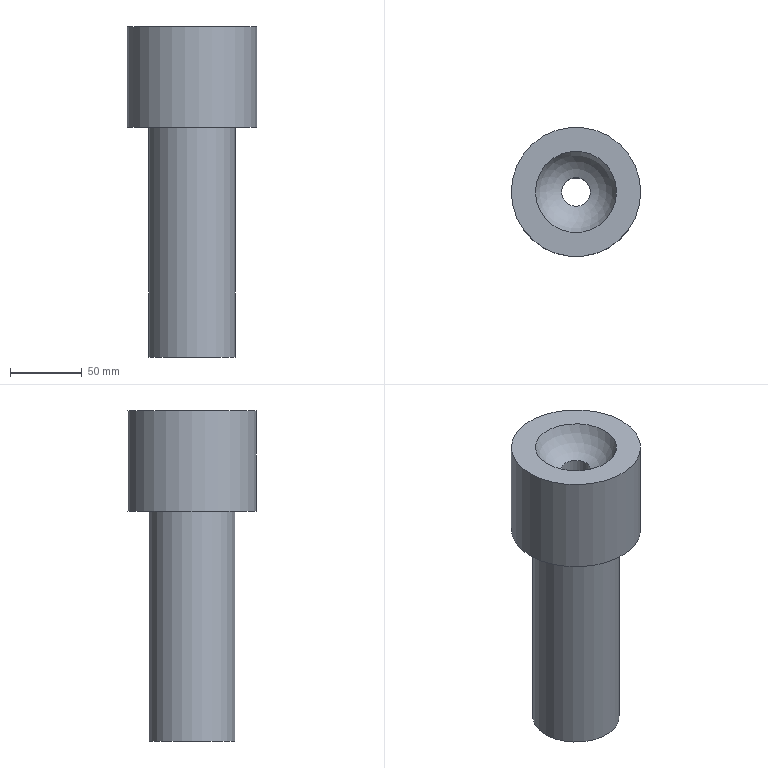Component | NX | BALL_SOCKET | 1 solid | 9 faces | box 90 x 90 x 230 mm | volume 786440 mm3 | cylinder 4 | plane 4 | sphere 1 | commonest cylinder face diameters 90 x1 60 x1 30 x1 20 x1
STEP:
#1=CARTESIAN_POINT('',(0.,0.,0.));
#2=DIRECTION('',(0.,0.,1.));
#3=DIRECTION('',(1.,0.,0.));
#4=AXIS2_PLACEMENT_3D('',#1,#2,#3);
#5=CARTESIAN_POINT('',(517.45,0.,143.));
#6=VERTEX_POINT('',#5);
#7=CARTESIAN_POINT('',(562.45,0.,143.));
#8=DIRECTION('',(0.,0.,-1.));
#9=DIRECTION('',(-1.,0.,0.));
#10=AXIS2_PLACEMENT_3D('',#7,#8,#9);
#11=CIRCLE('',#10,45.);
#12=CARTESIAN_POINT('',(562.45,0.,213.));
#13=DIRECTION('',(0.,0.,-1.));
#14=DIRECTION('',(-1.,0.,0.));
#15=AXIS2_PLACEMENT_3D('',#12,#13,#14);
#16=CYLINDRICAL_SURFACE('',#15,45.);
#17=CARTESIAN_POINT('',(0.,70.));
#18=DIRECTION('',(1.,0.));
#19=VECTOR('',#18,1.);
#20=LINE('',#17,#19);
#21=(GEOMETRIC_REPRESENTATION_CONTEXT(2)PARAMETRIC_REPRESENTATION_CONTEXT()REPRESENTATION_CONTEXT('',''));
#22=DEFINITIONAL_REPRESENTATION('',(#20),#21);
#23=PCURVE('',#16,#22);
#24=CARTESIAN_POINT('',(562.45,-45.,143.));
#25=DIRECTION('',(0.,0.,1.));
#26=DIRECTION('',(1.,0.,0.));
#27=AXIS2_PLACEMENT_3D('',#24,#25,#26);
#28=PLANE('',#27);
#29=CARTESIAN_POINT('',(-45.,45.));
#30=CARTESIAN_POINT('',(-45.,122.942));
#31=CARTESIAN_POINT('',(22.5,83.971));
#32=CARTESIAN_POINT('',(90.,45.));
#33=CARTESIAN_POINT('',(22.5,6.029));
#34=CARTESIAN_POINT('',(-45.,-32.942));
#35=CARTESIAN_POINT('',(-45.,45.));
#36=(BOUNDED_CURVE()B_SPLINE_CURVE(2,(#29,#30,#31,#32,#33,#34,#35),.UNSPECIFIED.,.T.,.F.)B_SPLINE_CURVE_WITH_KNOTS((1,2,2,2,2,1),(-2.094,0.,2.094,4.189,6.283,8.378),.UNSPECIFIED.)CURVE()GEOMETRIC_REPRESENTATION_ITEM()RATIONAL_B_SPLINE_CURVE((1.,0.5,1.,0.5,1.,0.5,1.))REPRESENTATION_ITEM(''));
#37=(GEOMETRIC_REPRESENTATION_CONTEXT(2)PARAMETRIC_REPRESENTATION_CONTEXT()REPRESENTATION_CONTEXT('',''));
#38=DEFINITIONAL_REPRESENTATION('',(#36),#37);
#39=PCURVE('',#28,#38);
#40=SURFACE_CURVE('',#11,(#23,#39),.PCURVE_S1.);
#41=EDGE_CURVE('',#6,#6,#40,.T.);
#42=ORIENTED_EDGE('',*,*,#41,.F.);
#43=CARTESIAN_POINT('',(517.45,0.,213.));
#44=VERTEX_POINT('',#43);
#45=CARTESIAN_POINT('',(517.45,-0.,213.));
#46=CARTESIAN_POINT('',(517.45,-0.,143.));
#47=B_SPLINE_CURVE_WITH_KNOTS('',1,(#45,#46),.UNSPECIFIED.,.F.,.F.,(2,2),(0.,70.),.PIECEWISE_BEZIER_KNOTS.);
#48=CARTESIAN_POINT('',(0.,0.));
#49=DIRECTION('',(0.,1.));
#50=VECTOR('',#49,1.);
#51=LINE('',#48,#50);
#52=(GEOMETRIC_REPRESENTATION_CONTEXT(2)PARAMETRIC_REPRESENTATION_CONTEXT()REPRESENTATION_CONTEXT('',''));
#53=DEFINITIONAL_REPRESENTATION('',(#51),#52);
#54=PCURVE('',#16,#53);
#55=CARTESIAN_POINT('',(6.283,0.));
#56=DIRECTION('',(0.,1.));
#57=VECTOR('',#56,1.);
#58=LINE('',#55,#57);
#59=(GEOMETRIC_REPRESENTATION_CONTEXT(2)PARAMETRIC_REPRESENTATION_CONTEXT()REPRESENTATION_CONTEXT('',''));
#60=DEFINITIONAL_REPRESENTATION('',(#58),#59);
#61=PCURVE('',#16,#60);
#62=SEAM_CURVE('',#47,(#54,#61),.PCURVE_S1.);
#63=EDGE_CURVE('',#44,#6,#62,.T.);
#64=ORIENTED_EDGE('',*,*,#63,.F.);
#65=CARTESIAN_POINT('',(562.45,0.,213.));
#66=DIRECTION('',(0.,0.,-1.));
#67=DIRECTION('',(-1.,0.,0.));
#68=AXIS2_PLACEMENT_3D('',#65,#66,#67);
#69=CIRCLE('',#68,45.);
#70=CARTESIAN_POINT('',(0.,0.));
#71=DIRECTION('',(1.,0.));
#72=VECTOR('',#71,1.);
#73=LINE('',#70,#72);
#74=(GEOMETRIC_REPRESENTATION_CONTEXT(2)PARAMETRIC_REPRESENTATION_CONTEXT()REPRESENTATION_CONTEXT('',''));
#75=DEFINITIONAL_REPRESENTATION('',(#73),#74);
#76=PCURVE('',#16,#75);
#77=CARTESIAN_POINT('',(562.45,-28.284,213.));
#78=DIRECTION('',(0.,0.,-1.));
#79=DIRECTION('',(-1.,0.,0.));
#80=AXIS2_PLACEMENT_3D('',#77,#78,#79);
#81=PLANE('',#80);
#82=CARTESIAN_POINT('',(0.,28.284));
#83=DIRECTION('',(1.,0.));
#84=AXIS2_PLACEMENT_2D('',#82,#83);
#85=CIRCLE('',#84,45.);
#86=(GEOMETRIC_REPRESENTATION_CONTEXT(2)PARAMETRIC_REPRESENTATION_CONTEXT()REPRESENTATION_CONTEXT('',''));
#87=DEFINITIONAL_REPRESENTATION('',(#85),#86);
#88=PCURVE('',#81,#87);
#89=SURFACE_CURVE('',#69,(#76,#88),.PCURVE_S1.);
#90=EDGE_CURVE('',#44,#44,#89,.T.);
#91=ORIENTED_EDGE('',*,*,#90,.T.);
#92=ORIENTED_EDGE('',*,*,#63,.T.);
#93=EDGE_LOOP('',(#42,#64,#91,#92));
#94=FACE_BOUND('',#93,.T.);
#95=ADVANCED_FACE('',(#94),#16,.T.);
#96=CARTESIAN_POINT('',(532.45,0.,143.));
#97=VERTEX_POINT('',#96);
#98=CARTESIAN_POINT('',(562.45,0.,143.));
#99=DIRECTION('',(0.,0.,-1.));
#100=DIRECTION('',(-1.,0.,0.));
#101=AXIS2_PLACEMENT_3D('',#98,#99,#100);
#102=CIRCLE('',#101,30.);
#103=CARTESIAN_POINT('',(-30.,45.));
#104=CARTESIAN_POINT('',(-30.,96.962));
#105=CARTESIAN_POINT('',(15.,70.981));
#106=CARTESIAN_POINT('',(60.,45.));
#107=CARTESIAN_POINT('',(15.,19.019));
#108=CARTESIAN_POINT('',(-30.,-6.962));
#109=CARTESIAN_POINT('',(-30.,45.));
#110=(BOUNDED_CURVE()B_SPLINE_CURVE(2,(#103,#104,#105,#106,#107,#108,#109),.UNSPECIFIED.,.T.,.F.)B_SPLINE_CURVE_WITH_KNOTS((1,2,2,2,2,1),(-2.094,0.,2.094,4.189,6.283,8.378),.UNSPECIFIED.)CURVE()GEOMETRIC_REPRESENTATION_ITEM()RATIONAL_B_SPLINE_CURVE((1.,0.5,1.,0.5,1.,0.5,1.))REPRESENTATION_ITEM(''));
#111=(GEOMETRIC_REPRESENTATION_CONTEXT(2)PARAMETRIC_REPRESENTATION_CONTEXT()REPRESENTATION_CONTEXT('',''));
#112=DEFINITIONAL_REPRESENTATION('',(#110),#111);
#113=PCURVE('',#28,#112);
#114=CARTESIAN_POINT('',(562.45,0.,213.));
#115=DIRECTION('',(0.,0.,-1.));
#116=DIRECTION('',(-1.,0.,0.));
#117=AXIS2_PLACEMENT_3D('',#114,#115,#116);
#118=CYLINDRICAL_SURFACE('',#117,30.);
#119=CARTESIAN_POINT('',(0.,70.));
#120=DIRECTION('',(1.,0.));
#121=VECTOR('',#120,1.);
#122=LINE('',#119,#121);
#123=(GEOMETRIC_REPRESENTATION_CONTEXT(2)PARAMETRIC_REPRESENTATION_CONTEXT()REPRESENTATION_CONTEXT('',''));
#124=DEFINITIONAL_REPRESENTATION('',(#122),#123);
#125=PCURVE('',#118,#124);
#126=SURFACE_CURVE('',#102,(#113,#125),.PCURVE_S1.);
#127=EDGE_CURVE('',#97,#97,#126,.T.);
#128=ORIENTED_EDGE('',*,*,#127,.F.);
#129=EDGE_LOOP('',(#128));
#130=FACE_BOUND('',#129,.T.);
#131=ORIENTED_EDGE('',*,*,#41,.T.);
#132=EDGE_LOOP('',(#131));
#133=FACE_BOUND('',#132,.T.);
#134=ADVANCED_FACE('',(#130,#133),#28,.F.);
#135=CARTESIAN_POINT('',(532.45,0.,-17.));
#136=VERTEX_POINT('',#135);
#137=CARTESIAN_POINT('',(562.45,0.,-17.));
#138=DIRECTION('',(0.,0.,-1.));
#139=DIRECTION('',(-1.,0.,0.));
#140=AXIS2_PLACEMENT_3D('',#137,#138,#139);
#141=CIRCLE('',#140,30.);
#142=CARTESIAN_POINT('',(0.,230.));
#143=DIRECTION('',(1.,0.));
#144=VECTOR('',#143,1.);
#145=LINE('',#142,#144);
#146=(GEOMETRIC_REPRESENTATION_CONTEXT(2)PARAMETRIC_REPRESENTATION_CONTEXT()REPRESENTATION_CONTEXT('',''));
#147=DEFINITIONAL_REPRESENTATION('',(#145),#146);
#148=PCURVE('',#118,#147);
#149=CARTESIAN_POINT('',(562.45,-30.,-17.));
#150=DIRECTION('',(0.,0.,1.));
#151=DIRECTION('',(1.,0.,0.));
#152=AXIS2_PLACEMENT_3D('',#149,#150,#151);
#153=PLANE('',#152);
#154=CARTESIAN_POINT('',(-30.,30.));
#155=CARTESIAN_POINT('',(-30.,81.962));
#156=CARTESIAN_POINT('',(15.,55.981));
#157=CARTESIAN_POINT('',(60.,30.));
#158=CARTESIAN_POINT('',(15.,4.019));
#159=CARTESIAN_POINT('',(-30.,-21.962));
#160=CARTESIAN_POINT('',(-30.,30.));
#161=(BOUNDED_CURVE()B_SPLINE_CURVE(2,(#154,#155,#156,#157,#158,#159,#160),.UNSPECIFIED.,.T.,.F.)B_SPLINE_CURVE_WITH_KNOTS((1,2,2,2,2,1),(-2.094,0.,2.094,4.189,6.283,8.378),.UNSPECIFIED.)CURVE()GEOMETRIC_REPRESENTATION_ITEM()RATIONAL_B_SPLINE_CURVE((1.,0.5,1.,0.5,1.,0.5,1.))REPRESENTATION_ITEM(''));
#162=(GEOMETRIC_REPRESENTATION_CONTEXT(2)PARAMETRIC_REPRESENTATION_CONTEXT()REPRESENTATION_CONTEXT('',''));
#163=DEFINITIONAL_REPRESENTATION('',(#161),#162);
#164=PCURVE('',#153,#163);
#165=SURFACE_CURVE('',#141,(#148,#164),.PCURVE_S1.);
#166=EDGE_CURVE('',#136,#136,#165,.T.);
#167=ORIENTED_EDGE('',*,*,#166,.F.);
#168=CARTESIAN_POINT('',(532.45,-0.,143.));
#169=CARTESIAN_POINT('',(532.45,-0.,-17.));
#170=B_SPLINE_CURVE_WITH_KNOTS('',1,(#168,#169),.UNSPECIFIED.,.F.,.F.,(2,2),(70.,230.),.PIECEWISE_BEZIER_KNOTS.);
#171=CARTESIAN_POINT('',(0.,0.));
#172=DIRECTION('',(0.,1.));
#173=VECTOR('',#172,1.);
#174=LINE('',#171,#173);
#175=(GEOMETRIC_REPRESENTATION_CONTEXT(2)PARAMETRIC_REPRESENTATION_CONTEXT()REPRESENTATION_CONTEXT('',''));
#176=DEFINITIONAL_REPRESENTATION('',(#174),#175);
#177=PCURVE('',#118,#176);
#178=CARTESIAN_POINT('',(6.283,0.));
#179=DIRECTION('',(0.,1.));
#180=VECTOR('',#179,1.);
#181=LINE('',#178,#180);
#182=(GEOMETRIC_REPRESENTATION_CONTEXT(2)PARAMETRIC_REPRESENTATION_CONTEXT()REPRESENTATION_CONTEXT('',''));
#183=DEFINITIONAL_REPRESENTATION('',(#181),#182);
#184=PCURVE('',#118,#183);
#185=SEAM_CURVE('',#170,(#177,#184),.PCURVE_S1.);
#186=EDGE_CURVE('',#97,#136,#185,.T.);
#187=ORIENTED_EDGE('',*,*,#186,.F.);
#188=ORIENTED_EDGE('',*,*,#127,.T.);
#189=ORIENTED_EDGE('',*,*,#186,.T.);
#190=EDGE_LOOP('',(#167,#187,#188,#189));
#191=FACE_BOUND('',#190,.T.);
#192=ADVANCED_FACE('',(#191),#118,.T.);
#193=CARTESIAN_POINT('',(547.45,0.,-17.));
#194=VERTEX_POINT('',#193);
#195=CARTESIAN_POINT('',(562.45,0.,-17.));
#196=DIRECTION('',(0.,0.,-1.));
#197=DIRECTION('',(-1.,0.,0.));
#198=AXIS2_PLACEMENT_3D('',#195,#196,#197);
#199=CIRCLE('',#198,15.);
#200=CARTESIAN_POINT('',(-15.,30.));
#201=CARTESIAN_POINT('',(-15.,55.981));
#202=CARTESIAN_POINT('',(7.5,42.99));
#203=CARTESIAN_POINT('',(30.,30.));
#204=CARTESIAN_POINT('',(7.5,17.01));
#205=CARTESIAN_POINT('',(-15.,4.019));
#206=CARTESIAN_POINT('',(-15.,30.));
#207=(BOUNDED_CURVE()B_SPLINE_CURVE(2,(#200,#201,#202,#203,#204,#205,#206),.UNSPECIFIED.,.T.,.F.)B_SPLINE_CURVE_WITH_KNOTS((1,2,2,2,2,1),(-2.094,0.,2.094,4.189,6.283,8.378),.UNSPECIFIED.)CURVE()GEOMETRIC_REPRESENTATION_ITEM()RATIONAL_B_SPLINE_CURVE((1.,0.5,1.,0.5,1.,0.5,1.))REPRESENTATION_ITEM(''));
#208=(GEOMETRIC_REPRESENTATION_CONTEXT(2)PARAMETRIC_REPRESENTATION_CONTEXT()REPRESENTATION_CONTEXT('',''));
#209=DEFINITIONAL_REPRESENTATION('',(#207),#208);
#210=PCURVE('',#153,#209);
#211=CARTESIAN_POINT('',(562.45,0.,213.));
#212=DIRECTION('',(0.,0.,-1.));
#213=DIRECTION('',(-1.,0.,0.));
#214=AXIS2_PLACEMENT_3D('',#211,#212,#213);
#215=CYLINDRICAL_SURFACE('',#214,15.);
#216=CARTESIAN_POINT('',(0.,230.));
#217=DIRECTION('',(1.,0.));
#218=VECTOR('',#217,1.);
#219=LINE('',#216,#218);
#220=(GEOMETRIC_REPRESENTATION_CONTEXT(2)PARAMETRIC_REPRESENTATION_CONTEXT()REPRESENTATION_CONTEXT('',''));
#221=DEFINITIONAL_REPRESENTATION('',(#219),#220);
#222=PCURVE('',#215,#221);
#223=SURFACE_CURVE('',#199,(#210,#222),.PCURVE_S1.);
#224=EDGE_CURVE('',#194,#194,#223,.T.);
#225=ORIENTED_EDGE('',*,*,#224,.F.);
#226=EDGE_LOOP('',(#225));
#227=FACE_BOUND('',#226,.T.);
#228=ORIENTED_EDGE('',*,*,#166,.T.);
#229=EDGE_LOOP('',(#228));
#230=FACE_BOUND('',#229,.T.);
#231=ADVANCED_FACE('',(#227,#230),#153,.F.);
#232=CARTESIAN_POINT('',(547.45,0.,23.));
#233=VERTEX_POINT('',#232);
#234=CARTESIAN_POINT('',(562.45,0.,23.));
#235=DIRECTION('',(0.,0.,-1.));
#236=DIRECTION('',(-1.,0.,0.));
#237=AXIS2_PLACEMENT_3D('',#234,#235,#236);
#238=CIRCLE('',#237,15.);
#239=CARTESIAN_POINT('',(0.,190.));
#240=DIRECTION('',(1.,0.));
#241=VECTOR('',#240,1.);
#242=LINE('',#239,#241);
#243=(GEOMETRIC_REPRESENTATION_CONTEXT(2)PARAMETRIC_REPRESENTATION_CONTEXT()REPRESENTATION_CONTEXT('',''));
#244=DEFINITIONAL_REPRESENTATION('',(#242),#243);
#245=PCURVE('',#215,#244);
#246=CARTESIAN_POINT('',(562.45,-15.,23.));
#247=DIRECTION('',(0.,0.,1.));
#248=DIRECTION('',(1.,0.,0.));
#249=AXIS2_PLACEMENT_3D('',#246,#247,#248);
#250=PLANE('',#249);
#251=CARTESIAN_POINT('',(-15.,15.));
#252=CARTESIAN_POINT('',(-15.,40.981));
#253=CARTESIAN_POINT('',(7.5,27.99));
#254=CARTESIAN_POINT('',(30.,15.));
#255=CARTESIAN_POINT('',(7.5,2.01));
#256=CARTESIAN_POINT('',(-15.,-10.981));
#257=CARTESIAN_POINT('',(-15.,15.));
#258=(BOUNDED_CURVE()B_SPLINE_CURVE(2,(#251,#252,#253,#254,#255,#256,#257),.UNSPECIFIED.,.T.,.F.)B_SPLINE_CURVE_WITH_KNOTS((1,2,2,2,2,1),(-2.094,0.,2.094,4.189,6.283,8.378),.UNSPECIFIED.)CURVE()GEOMETRIC_REPRESENTATION_ITEM()RATIONAL_B_SPLINE_CURVE((1.,0.5,1.,0.5,1.,0.5,1.))REPRESENTATION_ITEM(''));
#259=(GEOMETRIC_REPRESENTATION_CONTEXT(2)PARAMETRIC_REPRESENTATION_CONTEXT()REPRESENTATION_CONTEXT('',''));
#260=DEFINITIONAL_REPRESENTATION('',(#258),#259);
#261=PCURVE('',#250,#260);
#262=SURFACE_CURVE('',#238,(#245,#261),.PCURVE_S1.);
#263=EDGE_CURVE('',#233,#233,#262,.T.);
#264=ORIENTED_EDGE('',*,*,#263,.T.);
#265=CARTESIAN_POINT('',(547.45,0.,23.));
#266=CARTESIAN_POINT('',(547.45,0.,-17.));
#267=B_SPLINE_CURVE_WITH_KNOTS('',1,(#265,#266),.UNSPECIFIED.,.F.,.F.,(2,2),(190.,230.),.PIECEWISE_BEZIER_KNOTS.);
#268=CARTESIAN_POINT('',(6.283,0.));
#269=DIRECTION('',(0.,1.));
#270=VECTOR('',#269,1.);
#271=LINE('',#268,#270);
#272=(GEOMETRIC_REPRESENTATION_CONTEXT(2)PARAMETRIC_REPRESENTATION_CONTEXT()REPRESENTATION_CONTEXT('',''));
#273=DEFINITIONAL_REPRESENTATION('',(#271),#272);
#274=PCURVE('',#215,#273);
#275=CARTESIAN_POINT('',(0.,0.));
#276=DIRECTION('',(0.,1.));
#277=VECTOR('',#276,1.);
#278=LINE('',#275,#277);
#279=(GEOMETRIC_REPRESENTATION_CONTEXT(2)PARAMETRIC_REPRESENTATION_CONTEXT()REPRESENTATION_CONTEXT('',''));
#280=DEFINITIONAL_REPRESENTATION('',(#278),#279);
#281=PCURVE('',#215,#280);
#282=SEAM_CURVE('',#267,(#274,#281),.PCURVE_S1.);
#283=EDGE_CURVE('',#233,#194,#282,.T.);
#284=ORIENTED_EDGE('',*,*,#283,.T.);
#285=ORIENTED_EDGE('',*,*,#224,.F.);
#286=ORIENTED_EDGE('',*,*,#283,.F.);
#287=EDGE_LOOP('',(#264,#284,#285,#286));
#288=FACE_BOUND('',#287,.F.);
#289=ADVANCED_FACE('',(#288),#215,.F.);
#290=CARTESIAN_POINT('',(552.45,0.,23.));
#291=VERTEX_POINT('',#290);
#292=CARTESIAN_POINT('',(562.45,0.,23.));
#293=DIRECTION('',(0.,0.,-1.));
#294=DIRECTION('',(-1.,0.,0.));
#295=AXIS2_PLACEMENT_3D('',#292,#293,#294);
#296=CIRCLE('',#295,10.);
#297=CARTESIAN_POINT('',(-10.,15.));
#298=CARTESIAN_POINT('',(-10.,32.321));
#299=CARTESIAN_POINT('',(5.,23.66));
#300=CARTESIAN_POINT('',(20.,15.));
#301=CARTESIAN_POINT('',(5.,6.34));
#302=CARTESIAN_POINT('',(-10.,-2.321));
#303=CARTESIAN_POINT('',(-10.,15.));
#304=(BOUNDED_CURVE()B_SPLINE_CURVE(2,(#297,#298,#299,#300,#301,#302,#303),.UNSPECIFIED.,.T.,.F.)B_SPLINE_CURVE_WITH_KNOTS((1,2,2,2,2,1),(-2.094,0.,2.094,4.189,6.283,8.378),.UNSPECIFIED.)CURVE()GEOMETRIC_REPRESENTATION_ITEM()RATIONAL_B_SPLINE_CURVE((1.,0.5,1.,0.5,1.,0.5,1.))REPRESENTATION_ITEM(''));
#305=(GEOMETRIC_REPRESENTATION_CONTEXT(2)PARAMETRIC_REPRESENTATION_CONTEXT()REPRESENTATION_CONTEXT('',''));
#306=DEFINITIONAL_REPRESENTATION('',(#304),#305);
#307=PCURVE('',#250,#306);
#308=CARTESIAN_POINT('',(562.45,0.,213.));
#309=DIRECTION('',(0.,0.,-1.));
#310=DIRECTION('',(-1.,0.,0.));
#311=AXIS2_PLACEMENT_3D('',#308,#309,#310);
#312=CYLINDRICAL_SURFACE('',#311,10.);
#313=CARTESIAN_POINT('',(0.,190.));
#314=DIRECTION('',(1.,0.));
#315=VECTOR('',#314,1.);
#316=LINE('',#313,#315);
#317=(GEOMETRIC_REPRESENTATION_CONTEXT(2)PARAMETRIC_REPRESENTATION_CONTEXT()REPRESENTATION_CONTEXT('',''));
#318=DEFINITIONAL_REPRESENTATION('',(#316),#317);
#319=PCURVE('',#312,#318);
#320=SURFACE_CURVE('',#296,(#307,#319),.PCURVE_S1.);
#321=EDGE_CURVE('',#291,#291,#320,.T.);
#322=ORIENTED_EDGE('',*,*,#321,.F.);
#323=EDGE_LOOP('',(#322));
#324=FACE_BOUND('',#323,.T.);
#325=ORIENTED_EDGE('',*,*,#263,.T.);
#326=EDGE_LOOP('',(#325));
#327=FACE_BOUND('',#326,.T.);
#328=ADVANCED_FACE('',(#324,#327),#250,.F.);
#329=CARTESIAN_POINT('',(552.45,0.,194.716));
#330=VERTEX_POINT('',#329);
#331=CARTESIAN_POINT('',(562.45,0.,194.716));
#332=DIRECTION('',(0.,0.,-1.));
#333=DIRECTION('',(-1.,0.,0.));
#334=AXIS2_PLACEMENT_3D('',#331,#332,#333);
#335=CIRCLE('',#334,10.);
#336=CARTESIAN_POINT('',(0.,18.284));
#337=DIRECTION('',(1.,0.));
#338=VECTOR('',#337,1.);
#339=LINE('',#336,#338);
#340=(GEOMETRIC_REPRESENTATION_CONTEXT(2)PARAMETRIC_REPRESENTATION_CONTEXT()REPRESENTATION_CONTEXT('',''));
#341=DEFINITIONAL_REPRESENTATION('',(#339),#340);
#342=PCURVE('',#312,#341);
#343=CARTESIAN_POINT('',(562.45,0.,223.));
#344=DIRECTION('',(0.,-0.,-1.));
#345=DIRECTION('',(0.,-1.,0.));
#346=AXIS2_PLACEMENT_3D('',#343,#344,#345);
#347=SPHERICAL_SURFACE('',#346,30.);
#348=CARTESIAN_POINT('',(1.571,1.231));
#349=CARTESIAN_POINT('',(1.666,1.231));
#350=CARTESIAN_POINT('',(1.856,1.231));
#351=CARTESIAN_POINT('',(2.142,1.231));
#352=CARTESIAN_POINT('',(2.428,1.231));
#353=CARTESIAN_POINT('',(2.713,1.231));
#354=CARTESIAN_POINT('',(2.999,1.231));
#355=CARTESIAN_POINT('',(3.284,1.231));
#356=CARTESIAN_POINT('',(3.57,1.231));
#357=CARTESIAN_POINT('',(3.856,1.231));
#358=CARTESIAN_POINT('',(4.141,1.231));
#359=CARTESIAN_POINT('',(4.427,1.231));
#360=CARTESIAN_POINT('',(4.712,1.231));
#361=CARTESIAN_POINT('',(4.998,1.231));
#362=CARTESIAN_POINT('',(5.284,1.231));
#363=CARTESIAN_POINT('',(5.569,1.231));
#364=CARTESIAN_POINT('',(5.855,1.231));
#365=CARTESIAN_POINT('',(6.14,1.231));
#366=CARTESIAN_POINT('',(6.426,1.231));
#367=CARTESIAN_POINT('',(6.712,1.231));
#368=CARTESIAN_POINT('',(6.997,1.231));
#369=CARTESIAN_POINT('',(7.283,1.231));
#370=CARTESIAN_POINT('',(7.568,1.231));
#371=CARTESIAN_POINT('',(7.759,1.231));
#372=CARTESIAN_POINT('',(7.854,1.231));
#373=B_SPLINE_CURVE_WITH_KNOTS('',3,(#348,#349,#350,#351,#352,#353,#354,#355,#356,#357,#358,#359,#360,#361,#362,#363,#364,#365,#366,#367,#368,#369,#370,#371,#372),.UNSPECIFIED.,.F.,.F.,(4,1,1,1,1,1,1,1,1,1,1,1,1,1,1,1,1,1,1,1,1,1,4),(0.,0.2856,0.5712,0.8568,1.142,1.428,1.714,1.999,2.285,2.57,2.856,3.142,3.427,3.713,3.998,4.284,4.57,4.855,5.141,5.426,5.712,5.998,6.283),.QUASI_UNIFORM_KNOTS.);
#374=(GEOMETRIC_REPRESENTATION_CONTEXT(2)PARAMETRIC_REPRESENTATION_CONTEXT()REPRESENTATION_CONTEXT('',''));
#375=DEFINITIONAL_REPRESENTATION('',(#373),#374);
#376=PCURVE('',#347,#375);
#377=SURFACE_CURVE('',#335,(#342,#376),.PCURVE_S1.);
#378=EDGE_CURVE('',#330,#330,#377,.T.);
#379=ORIENTED_EDGE('',*,*,#378,.T.);
#380=CARTESIAN_POINT('',(552.45,0.,194.716));
#381=CARTESIAN_POINT('',(552.45,0.,23.));
#382=B_SPLINE_CURVE_WITH_KNOTS('',1,(#380,#381),.UNSPECIFIED.,.F.,.F.,(2,2),(18.284,190.),.PIECEWISE_BEZIER_KNOTS.);
#383=CARTESIAN_POINT('',(6.283,0.));
#384=DIRECTION('',(0.,1.));
#385=VECTOR('',#384,1.);
#386=LINE('',#383,#385);
#387=(GEOMETRIC_REPRESENTATION_CONTEXT(2)PARAMETRIC_REPRESENTATION_CONTEXT()REPRESENTATION_CONTEXT('',''));
#388=DEFINITIONAL_REPRESENTATION('',(#386),#387);
#389=PCURVE('',#312,#388);
#390=CARTESIAN_POINT('',(0.,0.));
#391=DIRECTION('',(0.,1.));
#392=VECTOR('',#391,1.);
#393=LINE('',#390,#392);
#394=(GEOMETRIC_REPRESENTATION_CONTEXT(2)PARAMETRIC_REPRESENTATION_CONTEXT()REPRESENTATION_CONTEXT('',''));
#395=DEFINITIONAL_REPRESENTATION('',(#393),#394);
#396=PCURVE('',#312,#395);
#397=SEAM_CURVE('',#382,(#389,#396),.PCURVE_S1.);
#398=EDGE_CURVE('',#330,#291,#397,.T.);
#399=ORIENTED_EDGE('',*,*,#398,.T.);
#400=ORIENTED_EDGE('',*,*,#321,.F.);
#401=ORIENTED_EDGE('',*,*,#398,.F.);
#402=EDGE_LOOP('',(#379,#399,#400,#401));
#403=FACE_BOUND('',#402,.F.);
#404=ADVANCED_FACE('',(#403),#312,.F.);
#405=CARTESIAN_POINT('',(534.165,0.,213.));
#406=VERTEX_POINT('',#405);
#407=CARTESIAN_POINT('',(562.45,0.,213.));
#408=DIRECTION('',(0.,0.,-1.));
#409=DIRECTION('',(-1.,0.,0.));
#410=AXIS2_PLACEMENT_3D('',#407,#408,#409);
#411=CIRCLE('',#410,28.284);
#412=CARTESIAN_POINT('',(1.571,0.3398));
#413=CARTESIAN_POINT('',(1.666,0.3398));
#414=CARTESIAN_POINT('',(1.856,0.3398));
#415=CARTESIAN_POINT('',(2.142,0.3398));
#416=CARTESIAN_POINT('',(2.428,0.3398));
#417=CARTESIAN_POINT('',(2.713,0.3398));
#418=CARTESIAN_POINT('',(2.999,0.3398));
#419=CARTESIAN_POINT('',(3.284,0.3398));
#420=CARTESIAN_POINT('',(3.57,0.3398));
#421=CARTESIAN_POINT('',(3.856,0.3398));
#422=CARTESIAN_POINT('',(4.141,0.3398));
#423=CARTESIAN_POINT('',(4.427,0.3398));
#424=CARTESIAN_POINT('',(4.712,0.3398));
#425=CARTESIAN_POINT('',(4.998,0.3398));
#426=CARTESIAN_POINT('',(5.284,0.3398));
#427=CARTESIAN_POINT('',(5.569,0.3398));
#428=CARTESIAN_POINT('',(5.855,0.3398));
#429=CARTESIAN_POINT('',(6.14,0.3398));
#430=CARTESIAN_POINT('',(6.426,0.3398));
#431=CARTESIAN_POINT('',(6.712,0.3398));
#432=CARTESIAN_POINT('',(6.997,0.3398));
#433=CARTESIAN_POINT('',(7.283,0.3398));
#434=CARTESIAN_POINT('',(7.568,0.3398));
#435=CARTESIAN_POINT('',(7.759,0.3398));
#436=CARTESIAN_POINT('',(7.854,0.3398));
#437=B_SPLINE_CURVE_WITH_KNOTS('',3,(#412,#413,#414,#415,#416,#417,#418,#419,#420,#421,#422,#423,#424,#425,#426,#427,#428,#429,#430,#431,#432,#433,#434,#435,#436),.UNSPECIFIED.,.F.,.F.,(4,1,1,1,1,1,1,1,1,1,1,1,1,1,1,1,1,1,1,1,1,1,4),(0.,0.2856,0.5712,0.8568,1.142,1.428,1.714,1.999,2.285,2.57,2.856,3.142,3.427,3.713,3.998,4.284,4.57,4.855,5.141,5.426,5.712,5.998,6.283),.QUASI_UNIFORM_KNOTS.);
#438=(GEOMETRIC_REPRESENTATION_CONTEXT(2)PARAMETRIC_REPRESENTATION_CONTEXT()REPRESENTATION_CONTEXT('',''));
#439=DEFINITIONAL_REPRESENTATION('',(#437),#438);
#440=PCURVE('',#347,#439);
#441=CARTESIAN_POINT('',(0.,28.284));
#442=DIRECTION('',(1.,0.));
#443=AXIS2_PLACEMENT_2D('',#441,#442);
#444=CIRCLE('',#443,28.284);
#445=(GEOMETRIC_REPRESENTATION_CONTEXT(2)PARAMETRIC_REPRESENTATION_CONTEXT()REPRESENTATION_CONTEXT('',''));
#446=DEFINITIONAL_REPRESENTATION('',(#444),#445);
#447=PCURVE('',#81,#446);
#448=SURFACE_CURVE('',#411,(#440,#447),.PCURVE_S1.);
#449=EDGE_CURVE('',#406,#406,#448,.T.);
#450=ORIENTED_EDGE('',*,*,#449,.T.);
#451=CARTESIAN_POINT('',(534.165,0.,213.));
#452=CARTESIAN_POINT('',(535.651,0.,208.799));
#453=CARTESIAN_POINT('',(537.884,0.,204.863));
#454=CARTESIAN_POINT('',(540.808,0.,201.358));
#455=CARTESIAN_POINT('',(544.313,0.,198.435));
#456=CARTESIAN_POINT('',(548.249,0.,196.201));
#457=CARTESIAN_POINT('',(552.45,0.,194.716));
#458=B_SPLINE_CURVE_WITH_KNOTS('',6,(#451,#452,#453,#454,#455,#456,#457),.UNSPECIFIED.,.F.,.F.,(7,7),(0.3398,1.231),.PIECEWISE_BEZIER_KNOTS.);
#459=CARTESIAN_POINT('',(7.854,0.));
#460=DIRECTION('',(0.,1.));
#461=VECTOR('',#460,1.);
#462=LINE('',#459,#461);
#463=(GEOMETRIC_REPRESENTATION_CONTEXT(2)PARAMETRIC_REPRESENTATION_CONTEXT()REPRESENTATION_CONTEXT('',''));
#464=DEFINITIONAL_REPRESENTATION('',(#462),#463);
#465=PCURVE('',#347,#464);
#466=CARTESIAN_POINT('',(1.571,0.));
#467=DIRECTION('',(0.,1.));
#468=VECTOR('',#467,1.);
#469=LINE('',#466,#468);
#470=(GEOMETRIC_REPRESENTATION_CONTEXT(2)PARAMETRIC_REPRESENTATION_CONTEXT()REPRESENTATION_CONTEXT('',''));
#471=DEFINITIONAL_REPRESENTATION('',(#469),#470);
#472=PCURVE('',#347,#471);
#473=SEAM_CURVE('',#458,(#465,#472),.PCURVE_S1.);
#474=EDGE_CURVE('',#406,#330,#473,.T.);
#475=ORIENTED_EDGE('',*,*,#474,.T.);
#476=ORIENTED_EDGE('',*,*,#378,.F.);
#477=ORIENTED_EDGE('',*,*,#474,.F.);
#478=EDGE_LOOP('',(#450,#475,#476,#477));
#479=FACE_BOUND('',#478,.F.);
#480=ADVANCED_FACE('',(#479),#347,.F.);
#481=ORIENTED_EDGE('',*,*,#90,.F.);
#482=EDGE_LOOP('',(#481));
#483=FACE_BOUND('',#482,.T.);
#484=ORIENTED_EDGE('',*,*,#449,.T.);
#485=EDGE_LOOP('',(#484));
#486=FACE_BOUND('',#485,.T.);
#487=ADVANCED_FACE('',(#483,#486),#81,.F.);
#488=CLOSED_SHELL('',(#95,#134,#192,#231,#289,#328,#404,#480,#487));
#489=MANIFOLD_SOLID_BREP('',#488);
#490=(LENGTH_UNIT()NAMED_UNIT(*)SI_UNIT(.MILLI.,.METRE.));
#491=UNCERTAINTY_MEASURE_WITH_UNIT(LENGTH_MEASURE(0.00001),#490,'','');
#492=(NAMED_UNIT(*)PLANE_ANGLE_UNIT()SI_UNIT($,.RADIAN.));
#493=(NAMED_UNIT(*)SI_UNIT($,.STERADIAN.)SOLID_ANGLE_UNIT());
#494=(GEOMETRIC_REPRESENTATION_CONTEXT(3)GLOBAL_UNCERTAINTY_ASSIGNED_CONTEXT((#491))GLOBAL_UNIT_ASSIGNED_CONTEXT((#490,#492,#493))REPRESENTATION_CONTEXT('',''));
#495=ADVANCED_BREP_SHAPE_REPRESENTATION('',(#4,#489),#494);